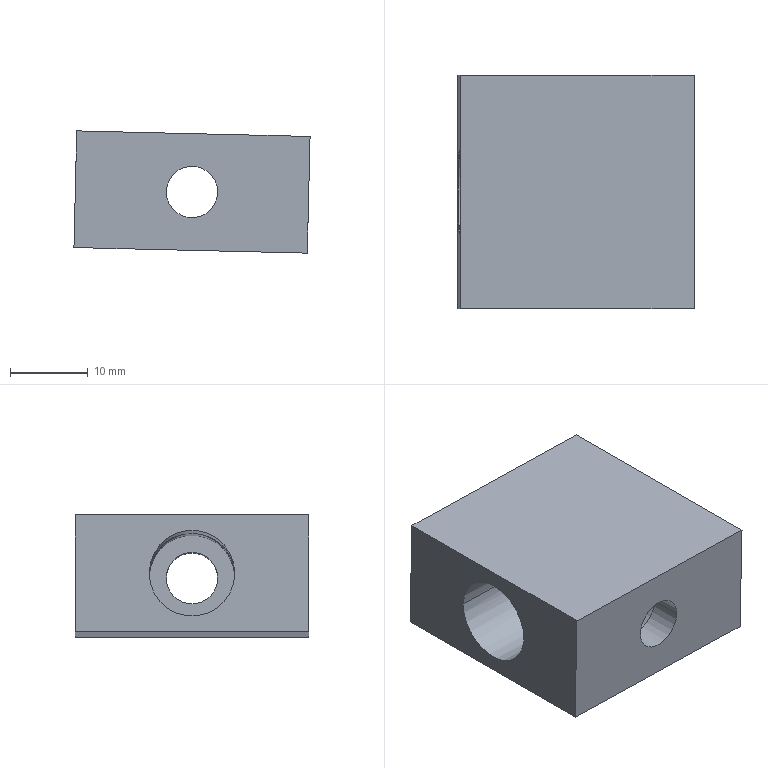Component | SolidWorks | 2012MB0201-1_ASideDoor-1-1_1530ConnectorAMS12-1530-5 | 1 solid | 20 faces | box 30.35 x 30 x 15.71 mm | volume 9172 mm3 | cylinder 12 | plane 8 | commonest cylinder face diameters 11 x8 6.6 x4
build123d program:
from build123d import *

# Parameters (mm, degrees)
SKETCH1_W                                            = 30
SKETCH1_H                                            = 30
BOSS_EXTRUDE1_DEPTH                                  = 15
M6_HEX_SOCKET_HEAD_CAP_SCREW_COUNTERBORE_D           = 6.6
M6_HEX_SOCKET_HEAD_CAP_SCREW_COUNTERBORE_CBORE_D     = 11
M6_HEX_SOCKET_HEAD_CAP_SCREW_COUNTERBORE_CBORE_DEPTH = 26
M6_HEX_SOCKET_HEAD_CAP_SCREW_COUNTER_2_D             = 6.6
M6_HEX_SOCKET_HEAD_CAP_SCREW_COUNTER_2_CBORE_D       = 11
M6_HEX_SOCKET_HEAD_CAP_SCREW_COUNTER_2_CBORE_DEPTH   = 26


with BuildPart() as part:
    # Sketch1 → Boss-Extrude1 (new body)
    with BuildSketch(Plane(origin=(0, 0, 0), x_dir=(1, 0, 0), z_dir=(0, 1, 0))):
        Rectangle(SKETCH1_W, SKETCH1_H)
    extrude(amount=BOSS_EXTRUDE1_DEPTH)

    # M6 Hex Socket Head Cap Screw Counterbore (through all)
    with Locations(Plane(origin=(-15, 7.5, 0), x_dir=(0, 0, -1), z_dir=(-1, 0, 0))):
        with Locations((0, 0)):
            CounterBoreHole(M6_HEX_SOCKET_HEAD_CAP_SCREW_COUNTERBORE_D / 2, M6_HEX_SOCKET_HEAD_CAP_SCREW_COUNTERBORE_CBORE_D / 2, M6_HEX_SOCKET_HEAD_CAP_SCREW_COUNTERBORE_CBORE_DEPTH)

    # M6 Hex Socket Head Cap Screw Counter 2 (through all)
    with Locations(Plane(origin=(0, 7.5, -15), x_dir=(-1, 0, 0), z_dir=(0, 0, -1))):
        with Locations((0, 0)):
            CounterBoreHole(M6_HEX_SOCKET_HEAD_CAP_SCREW_COUNTER_2_D / 2, M6_HEX_SOCKET_HEAD_CAP_SCREW_COUNTER_2_CBORE_D / 2, M6_HEX_SOCKET_HEAD_CAP_SCREW_COUNTER_2_CBORE_DEPTH)


solid = part.part

# Placed as in the assembly
solid = solid.moved(Location((-1264.623, 987.35, -171.755), (-180, 88.629, 90)))
STEP:
#1=COLOUR_RGB('',0.7922,0.8196,0.9333);
#2=FILL_AREA_STYLE_COLOUR('',#1);
#3=FILL_AREA_STYLE('',(#2));
#4=SURFACE_STYLE_FILL_AREA(#3);
#5=SURFACE_SIDE_STYLE('',(#4));
#6=SURFACE_STYLE_USAGE(.BOTH.,#5);
#7=PRESENTATION_STYLE_ASSIGNMENT((#6));
#8=CARTESIAN_POINT('',(-49.205,39.002,-7.071));
#9=VERTEX_POINT('',#8);
#10=CARTESIAN_POINT('',(-49.205,38.742,-7.071));
#11=VERTEX_POINT('',#10);
#12=CARTESIAN_POINT('',(-49.205,38.872,-7.071));
#13=DIRECTION('',(-0.9997,-0.,0.02392));
#14=DIRECTION('',(0.,-1.,0.));
#15=AXIS2_PLACEMENT_3D('',#12,#13,#14);
#16=CIRCLE('',#15,0.1299);
#17=EDGE_CURVE('',#9,#11,#16,.T.);
#18=ORIENTED_EDGE('',*,*,#17,.F.);
#19=CARTESIAN_POINT('',(-49.362,39.002,-7.068));
#20=VERTEX_POINT('',#19);
#21=CARTESIAN_POINT('',(-50.386,39.002,-7.043));
#22=DIRECTION('',(-0.9997,-0.,0.02392));
#23=VECTOR('',#22,39.37);
#24=LINE('',#21,#23);
#25=EDGE_CURVE('',#9,#20,#24,.T.);
#26=ORIENTED_EDGE('',*,*,#25,.T.);
#27=CARTESIAN_POINT('',(-49.362,38.742,-7.068));
#28=VERTEX_POINT('',#27);
#29=CARTESIAN_POINT('',(-49.362,38.872,-7.068));
#30=DIRECTION('',(-0.9997,-0.,0.02392));
#31=DIRECTION('',(0.,-1.,0.));
#32=AXIS2_PLACEMENT_3D('',#29,#30,#31);
#33=CIRCLE('',#32,0.1299);
#34=EDGE_CURVE('',#20,#28,#33,.T.);
#35=ORIENTED_EDGE('',*,*,#34,.T.);
#36=CARTESIAN_POINT('',(-50.386,38.742,-7.043));
#37=DIRECTION('',(-0.9997,-0.,0.02392));
#38=VECTOR('',#37,39.37);
#39=LINE('',#36,#38);
#40=EDGE_CURVE('',#11,#28,#39,.T.);
#41=ORIENTED_EDGE('',*,*,#40,.F.);
#42=EDGE_LOOP('',(#18,#26,#35,#41));
#43=FACE_OUTER_BOUND('',#42,.T.);
#44=CARTESIAN_POINT('',(-50.386,38.872,-7.043));
#45=DIRECTION('',(-0.9997,-0.,0.02392));
#46=DIRECTION('',(0.,-1.,0.));
#47=AXIS2_PLACEMENT_3D('',#44,#45,#46);
#48=CYLINDRICAL_SURFACE('',#47,0.1299);
#49=ADVANCED_FACE('',(#43),#48,.F.);
#50=CARTESIAN_POINT('',(-49.362,39.089,-7.068));
#51=VERTEX_POINT('',#50);
#52=CARTESIAN_POINT('',(-49.362,38.656,-7.068));
#53=VERTEX_POINT('',#52);
#54=CARTESIAN_POINT('',(-49.362,38.872,-7.068));
#55=DIRECTION('',(-0.9997,-0.,0.02392));
#56=DIRECTION('',(0.,-1.,0.));
#57=AXIS2_PLACEMENT_3D('',#54,#55,#56);
#58=CIRCLE('',#57,0.2165);
#59=EDGE_CURVE('',#51,#53,#58,.T.);
#60=ORIENTED_EDGE('',*,*,#59,.F.);
#61=CARTESIAN_POINT('',(-49.579,39.089,-7.062));
#62=VERTEX_POINT('',#61);
#63=CARTESIAN_POINT('',(-50.386,39.089,-7.043));
#64=DIRECTION('',(-0.9997,-0.,0.02392));
#65=VECTOR('',#64,39.37);
#66=LINE('',#63,#65);
#67=EDGE_CURVE('',#51,#62,#66,.T.);
#68=ORIENTED_EDGE('',*,*,#67,.T.);
#69=CARTESIAN_POINT('',(-49.801,38.872,-7.274));
#70=VERTEX_POINT('',#69);
#71=CARTESIAN_POINT('',(-49.801,38.872,-7.274));
#72=CARTESIAN_POINT('',(-49.674,38.999,-7.277));
#73=CARTESIAN_POINT('',(-49.582,39.089,-7.189));
#74=CARTESIAN_POINT('',(-49.579,39.089,-7.062));
#75=(BOUNDED_CURVE()B_SPLINE_CURVE(3,(#71,#72,#73,#74),.UNSPECIFIED.,.F.,.T.)B_SPLINE_CURVE_WITH_KNOTS((4,4),(4.712,6.283),.UNSPECIFIED.)CURVE()GEOMETRIC_REPRESENTATION_ITEM()RATIONAL_B_SPLINE_CURVE((1.,0.8047,0.8047,1.))REPRESENTATION_ITEM(''));
#76=EDGE_CURVE('',#70,#62,#75,.T.);
#77=ORIENTED_EDGE('',*,*,#76,.F.);
#78=CARTESIAN_POINT('',(-49.579,38.656,-7.062));
#79=VERTEX_POINT('',#78);
#80=CARTESIAN_POINT('',(-49.579,38.656,-7.062));
#81=CARTESIAN_POINT('',(-49.582,38.656,-7.189));
#82=CARTESIAN_POINT('',(-49.674,38.745,-7.277));
#83=CARTESIAN_POINT('',(-49.801,38.872,-7.274));
#84=(BOUNDED_CURVE()B_SPLINE_CURVE(3,(#80,#81,#82,#83),.UNSPECIFIED.,.F.,.F.)B_SPLINE_CURVE_WITH_KNOTS((4,4),(3.142,4.712),.UNSPECIFIED.)CURVE()GEOMETRIC_REPRESENTATION_ITEM()RATIONAL_B_SPLINE_CURVE((1.,0.8047,0.8047,1.))REPRESENTATION_ITEM(''));
#85=EDGE_CURVE('',#79,#70,#84,.T.);
#86=ORIENTED_EDGE('',*,*,#85,.F.);
#87=CARTESIAN_POINT('',(-50.386,38.656,-7.043));
#88=DIRECTION('',(-0.9997,-0.,0.02392));
#89=VECTOR('',#88,39.37);
#90=LINE('',#87,#89);
#91=EDGE_CURVE('',#53,#79,#90,.T.);
#92=ORIENTED_EDGE('',*,*,#91,.F.);
#93=EDGE_LOOP('',(#60,#68,#77,#86,#92));
#94=FACE_OUTER_BOUND('',#93,.T.);
#95=CARTESIAN_POINT('',(-50.386,38.872,-7.043));
#96=DIRECTION('',(-0.9997,-0.,0.02392));
#97=DIRECTION('',(0.,-1.,0.));
#98=AXIS2_PLACEMENT_3D('',#95,#96,#97);
#99=CYLINDRICAL_SURFACE('',#98,0.2165);
#100=ADVANCED_FACE('',(#94),#99,.F.);
#101=CARTESIAN_POINT('',(-50.012,39.089,-7.052));
#102=VERTEX_POINT('',#101);
#103=CARTESIAN_POINT('',(-50.012,39.089,-7.052));
#104=CARTESIAN_POINT('',(-50.015,39.089,-7.179));
#105=CARTESIAN_POINT('',(-49.927,38.999,-7.271));
#106=CARTESIAN_POINT('',(-49.801,38.872,-7.274));
#107=(BOUNDED_CURVE()B_SPLINE_CURVE(3,(#103,#104,#105,#106),.UNSPECIFIED.,.F.,.F.)B_SPLINE_CURVE_WITH_KNOTS((4,4),(0.,1.571),.UNSPECIFIED.)CURVE()GEOMETRIC_REPRESENTATION_ITEM()RATIONAL_B_SPLINE_CURVE((1.,0.8047,0.8047,1.))REPRESENTATION_ITEM(''));
#108=EDGE_CURVE('',#102,#70,#107,.T.);
#109=ORIENTED_EDGE('',*,*,#108,.F.);
#110=CARTESIAN_POINT('',(-50.386,39.089,-7.043));
#111=VERTEX_POINT('',#110);
#112=CARTESIAN_POINT('',(-50.386,39.089,-7.043));
#113=DIRECTION('',(-0.9997,-0.,0.02392));
#114=VECTOR('',#113,39.37);
#115=LINE('',#112,#114);
#116=EDGE_CURVE('',#102,#111,#115,.T.);
#117=ORIENTED_EDGE('',*,*,#116,.T.);
#118=CARTESIAN_POINT('',(-50.386,38.656,-7.043));
#119=VERTEX_POINT('',#118);
#120=CARTESIAN_POINT('',(-50.386,38.872,-7.043));
#121=DIRECTION('',(-0.9997,-0.,0.02392));
#122=DIRECTION('',(0.,-1.,0.));
#123=AXIS2_PLACEMENT_3D('',#120,#121,#122);
#124=CIRCLE('',#123,0.2165);
#125=EDGE_CURVE('',#111,#119,#124,.T.);
#126=ORIENTED_EDGE('',*,*,#125,.T.);
#127=CARTESIAN_POINT('',(-50.012,38.656,-7.052));
#128=VERTEX_POINT('',#127);
#129=CARTESIAN_POINT('',(-50.386,38.656,-7.043));
#130=DIRECTION('',(-0.9997,-0.,0.02392));
#131=VECTOR('',#130,39.37);
#132=LINE('',#129,#131);
#133=EDGE_CURVE('',#128,#119,#132,.T.);
#134=ORIENTED_EDGE('',*,*,#133,.F.);
#135=CARTESIAN_POINT('',(-49.801,38.872,-7.274));
#136=CARTESIAN_POINT('',(-49.927,38.745,-7.271));
#137=CARTESIAN_POINT('',(-50.015,38.656,-7.179));
#138=CARTESIAN_POINT('',(-50.012,38.656,-7.052));
#139=(BOUNDED_CURVE()B_SPLINE_CURVE(3,(#135,#136,#137,#138),.UNSPECIFIED.,.F.,.F.)B_SPLINE_CURVE_WITH_KNOTS((4,4),(1.571,3.142),.UNSPECIFIED.)CURVE()GEOMETRIC_REPRESENTATION_ITEM()RATIONAL_B_SPLINE_CURVE((1.,0.8047,0.8047,1.))REPRESENTATION_ITEM(''));
#140=EDGE_CURVE('',#70,#128,#139,.T.);
#141=ORIENTED_EDGE('',*,*,#140,.F.);
#142=EDGE_LOOP('',(#109,#117,#126,#134,#141));
#143=FACE_OUTER_BOUND('',#142,.T.);
#144=CARTESIAN_POINT('',(-50.386,38.872,-7.043));
#145=DIRECTION('',(-0.9997,-0.,0.02392));
#146=DIRECTION('',(0.,-1.,0.));
#147=AXIS2_PLACEMENT_3D('',#144,#145,#146);
#148=CYLINDRICAL_SURFACE('',#147,0.2165);
#149=ADVANCED_FACE('',(#143),#148,.F.);
#150=CARTESIAN_POINT('',(-49.579,38.439,-7.062));
#151=VERTEX_POINT('',#150);
#152=CARTESIAN_POINT('',(-50.012,38.439,-7.052));
#153=VERTEX_POINT('',#152);
#154=CARTESIAN_POINT('',(-49.795,38.439,-7.057));
#155=DIRECTION('',(-0.,1.,0.));
#156=DIRECTION('',(-0.9997,-0.,0.02392));
#157=AXIS2_PLACEMENT_3D('',#154,#155,#156);
#158=CIRCLE('',#157,0.2165);
#159=EDGE_CURVE('',#151,#153,#158,.T.);
#160=ORIENTED_EDGE('',*,*,#159,.F.);
#161=CARTESIAN_POINT('',(-49.579,39.463,-7.062));
#162=DIRECTION('',(-0.,1.,0.));
#163=VECTOR('',#162,39.37);
#164=LINE('',#161,#163);
#165=EDGE_CURVE('',#151,#79,#164,.T.);
#166=ORIENTED_EDGE('',*,*,#165,.T.);
#167=ORIENTED_EDGE('',*,*,#85,.T.);
#168=ORIENTED_EDGE('',*,*,#140,.T.);
#169=CARTESIAN_POINT('',(-50.012,39.463,-7.052));
#170=DIRECTION('',(-0.,1.,0.));
#171=VECTOR('',#170,39.37);
#172=LINE('',#169,#171);
#173=EDGE_CURVE('',#153,#128,#172,.T.);
#174=ORIENTED_EDGE('',*,*,#173,.F.);
#175=EDGE_LOOP('',(#160,#166,#167,#168,#174));
#176=FACE_OUTER_BOUND('',#175,.T.);
#177=CARTESIAN_POINT('',(-49.795,39.463,-7.057));
#178=DIRECTION('',(-0.,1.,0.));
#179=DIRECTION('',(-0.9997,0.,0.02392));
#180=AXIS2_PLACEMENT_3D('',#177,#178,#179);
#181=CYLINDRICAL_SURFACE('',#180,0.2165);
#182=ADVANCED_FACE('',(#176),#181,.F.);
#183=CARTESIAN_POINT('',(-49.666,38.282,-7.06));
#184=VERTEX_POINT('',#183);
#185=CARTESIAN_POINT('',(-49.925,38.282,-7.054));
#186=VERTEX_POINT('',#185);
#187=CARTESIAN_POINT('',(-49.795,38.282,-7.057));
#188=DIRECTION('',(-0.,1.,0.));
#189=DIRECTION('',(-0.9997,0.,0.02392));
#190=AXIS2_PLACEMENT_3D('',#187,#188,#189);
#191=CIRCLE('',#190,0.1299);
#192=EDGE_CURVE('',#184,#186,#191,.T.);
#193=ORIENTED_EDGE('',*,*,#192,.F.);
#194=CARTESIAN_POINT('',(-49.666,38.439,-7.06));
#195=VERTEX_POINT('',#194);
#196=CARTESIAN_POINT('',(-49.666,39.463,-7.06));
#197=DIRECTION('',(-0.,1.,0.));
#198=VECTOR('',#197,39.37);
#199=LINE('',#196,#198);
#200=EDGE_CURVE('',#184,#195,#199,.T.);
#201=ORIENTED_EDGE('',*,*,#200,.T.);
#202=CARTESIAN_POINT('',(-49.925,38.439,-7.054));
#203=VERTEX_POINT('',#202);
#204=CARTESIAN_POINT('',(-49.795,38.439,-7.057));
#205=DIRECTION('',(-0.,1.,0.));
#206=DIRECTION('',(-0.9997,0.,0.02392));
#207=AXIS2_PLACEMENT_3D('',#204,#205,#206);
#208=CIRCLE('',#207,0.1299);
#209=EDGE_CURVE('',#195,#203,#208,.T.);
#210=ORIENTED_EDGE('',*,*,#209,.T.);
#211=CARTESIAN_POINT('',(-49.925,39.463,-7.054));
#212=DIRECTION('',(-0.,1.,0.));
#213=VECTOR('',#212,39.37);
#214=LINE('',#211,#213);
#215=EDGE_CURVE('',#186,#203,#214,.T.);
#216=ORIENTED_EDGE('',*,*,#215,.F.);
#217=EDGE_LOOP('',(#193,#201,#210,#216));
#218=FACE_OUTER_BOUND('',#217,.T.);
#219=CARTESIAN_POINT('',(-49.795,39.463,-7.057));
#220=DIRECTION('',(-0.,1.,0.));
#221=DIRECTION('',(-0.9997,0.,0.02392));
#222=AXIS2_PLACEMENT_3D('',#219,#220,#221);
#223=CYLINDRICAL_SURFACE('',#222,0.1299);
#224=ADVANCED_FACE('',(#218),#223,.F.);
#225=ORIENTED_EDGE('',*,*,#76,.T.);
#226=CARTESIAN_POINT('',(-49.579,39.463,-7.062));
#227=VERTEX_POINT('',#226);
#228=CARTESIAN_POINT('',(-49.579,39.463,-7.062));
#229=DIRECTION('',(-0.,1.,0.));
#230=VECTOR('',#229,39.37);
#231=LINE('',#228,#230);
#232=EDGE_CURVE('',#62,#227,#231,.T.);
#233=ORIENTED_EDGE('',*,*,#232,.T.);
#234=CARTESIAN_POINT('',(-50.012,39.463,-7.052));
#235=VERTEX_POINT('',#234);
#236=CARTESIAN_POINT('',(-49.795,39.463,-7.057));
#237=DIRECTION('',(-0.,1.,0.));
#238=DIRECTION('',(-0.9997,0.,0.02392));
#239=AXIS2_PLACEMENT_3D('',#236,#237,#238);
#240=CIRCLE('',#239,0.2165);
#241=EDGE_CURVE('',#227,#235,#240,.T.);
#242=ORIENTED_EDGE('',*,*,#241,.T.);
#243=CARTESIAN_POINT('',(-50.012,39.463,-7.052));
#244=DIRECTION('',(-0.,1.,0.));
#245=VECTOR('',#244,39.37);
#246=LINE('',#243,#245);
#247=EDGE_CURVE('',#102,#235,#246,.T.);
#248=ORIENTED_EDGE('',*,*,#247,.F.);
#249=ORIENTED_EDGE('',*,*,#108,.T.);
#250=EDGE_LOOP('',(#225,#233,#242,#248,#249));
#251=FACE_OUTER_BOUND('',#250,.T.);
#252=CARTESIAN_POINT('',(-49.795,39.463,-7.057));
#253=DIRECTION('',(-0.,1.,0.));
#254=DIRECTION('',(-0.9997,0.,0.02392));
#255=AXIS2_PLACEMENT_3D('',#252,#253,#254);
#256=CYLINDRICAL_SURFACE('',#255,0.2165);
#257=ADVANCED_FACE('',(#251),#256,.F.);
#258=ORIENTED_EDGE('',*,*,#232,.F.);
#259=CARTESIAN_POINT('',(-49.79,38.872,-6.841));
#260=VERTEX_POINT('',#259);
#261=CARTESIAN_POINT('',(-49.579,39.089,-7.062));
#262=CARTESIAN_POINT('',(-49.576,39.089,-6.936));
#263=CARTESIAN_POINT('',(-49.663,38.999,-6.844));
#264=CARTESIAN_POINT('',(-49.79,38.872,-6.841));
#265=(BOUNDED_CURVE()B_SPLINE_CURVE(3,(#261,#262,#263,#264),.UNSPECIFIED.,.F.,.F.)B_SPLINE_CURVE_WITH_KNOTS((4,4),(0.,1.571),.UNSPECIFIED.)CURVE()GEOMETRIC_REPRESENTATION_ITEM()RATIONAL_B_SPLINE_CURVE((1.,0.8047,0.8047,1.))REPRESENTATION_ITEM(''));
#266=EDGE_CURVE('',#62,#260,#265,.T.);
#267=ORIENTED_EDGE('',*,*,#266,.T.);
#268=CARTESIAN_POINT('',(-49.79,38.872,-6.841));
#269=CARTESIAN_POINT('',(-49.917,38.999,-6.838));
#270=CARTESIAN_POINT('',(-50.009,39.089,-6.925));
#271=CARTESIAN_POINT('',(-50.012,39.089,-7.052));
#272=(BOUNDED_CURVE()B_SPLINE_CURVE(3,(#268,#269,#270,#271),.UNSPECIFIED.,.F.,.F.)B_SPLINE_CURVE_WITH_KNOTS((4,4),(4.712,6.283),.UNSPECIFIED.)CURVE()GEOMETRIC_REPRESENTATION_ITEM()RATIONAL_B_SPLINE_CURVE((1.,0.8047,0.8047,1.))REPRESENTATION_ITEM(''));
#273=EDGE_CURVE('',#260,#102,#272,.T.);
#274=ORIENTED_EDGE('',*,*,#273,.T.);
#275=ORIENTED_EDGE('',*,*,#247,.T.);
#276=CARTESIAN_POINT('',(-49.795,39.463,-7.057));
#277=DIRECTION('',(-0.,1.,0.));
#278=DIRECTION('',(-0.9997,0.,0.02392));
#279=AXIS2_PLACEMENT_3D('',#276,#277,#278);
#280=CIRCLE('',#279,0.2165);
#281=EDGE_CURVE('',#235,#227,#280,.T.);
#282=ORIENTED_EDGE('',*,*,#281,.T.);
#283=EDGE_LOOP('',(#258,#267,#274,#275,#282));
#284=FACE_OUTER_BOUND('',#283,.T.);
#285=CARTESIAN_POINT('',(-49.795,39.463,-7.057));
#286=DIRECTION('',(-0.,1.,0.));
#287=DIRECTION('',(-0.9997,0.,0.02392));
#288=AXIS2_PLACEMENT_3D('',#285,#286,#287);
#289=CYLINDRICAL_SURFACE('',#288,0.2165);
#290=ADVANCED_FACE('',(#284),#289,.F.);
#291=CARTESIAN_POINT('',(-49.205,38.872,-7.071));
#292=DIRECTION('',(-0.9997,-0.,0.02392));
#293=DIRECTION('',(0.,-1.,0.));
#294=AXIS2_PLACEMENT_3D('',#291,#292,#293);
#295=CIRCLE('',#294,0.1299);
#296=EDGE_CURVE('',#11,#9,#295,.T.);
#297=ORIENTED_EDGE('',*,*,#296,.T.);
#298=ORIENTED_EDGE('',*,*,#17,.T.);
#299=EDGE_LOOP('',(#297,#298));
#300=FACE_BOUND('',#299,.T.);
#301=CARTESIAN_POINT('',(-49.212,38.282,-7.367));
#302=VERTEX_POINT('',#301);
#303=CARTESIAN_POINT('',(-49.212,39.463,-7.367));
#304=VERTEX_POINT('',#303);
#305=CARTESIAN_POINT('',(-49.212,39.463,-7.367));
#306=DIRECTION('',(-0.,1.,0.));
#307=VECTOR('',#306,39.37);
#308=LINE('',#305,#307);
#309=EDGE_CURVE('',#302,#304,#308,.T.);
#310=ORIENTED_EDGE('',*,*,#309,.T.);
#311=CARTESIAN_POINT('',(-49.198,39.463,-6.776));
#312=VERTEX_POINT('',#311);
#313=CARTESIAN_POINT('',(-49.198,39.463,-6.776));
#314=DIRECTION('',(-0.02392,0.,-0.9997));
#315=VECTOR('',#314,39.37);
#316=LINE('',#313,#315);
#317=EDGE_CURVE('',#312,#304,#316,.T.);
#318=ORIENTED_EDGE('',*,*,#317,.F.);
#319=CARTESIAN_POINT('',(-49.198,38.282,-6.776));
#320=VERTEX_POINT('',#319);
#321=CARTESIAN_POINT('',(-49.198,39.463,-6.776));
#322=DIRECTION('',(-0.,1.,0.));
#323=VECTOR('',#322,39.37);
#324=LINE('',#321,#323);
#325=EDGE_CURVE('',#320,#312,#324,.T.);
#326=ORIENTED_EDGE('',*,*,#325,.F.);
#327=CARTESIAN_POINT('',(-49.198,38.282,-6.776));
#328=DIRECTION('',(-0.02392,0.,-0.9997));
#329=VECTOR('',#328,39.37);
#330=LINE('',#327,#329);
#331=EDGE_CURVE('',#320,#302,#330,.T.);
#332=ORIENTED_EDGE('',*,*,#331,.T.);
#333=EDGE_LOOP('',(#310,#318,#326,#332));
#334=FACE_OUTER_BOUND('',#333,.T.);
#335=CARTESIAN_POINT('',(-49.198,39.463,-6.776));
#336=DIRECTION('',(-0.9997,-0.,0.02392));
#337=DIRECTION('',(0.,-1.,-0.));
#338=AXIS2_PLACEMENT_3D('',#335,#336,#337);
#339=PLANE('',#338);
#340=ADVANCED_FACE('',(#300,#334),#339,.F.);
#341=ORIENTED_EDGE('',*,*,#281,.F.);
#342=ORIENTED_EDGE('',*,*,#241,.F.);
#343=EDGE_LOOP('',(#341,#342));
#344=FACE_BOUND('',#343,.T.);
#345=CARTESIAN_POINT('',(-50.393,39.463,-7.338));
#346=VERTEX_POINT('',#345);
#347=CARTESIAN_POINT('',(-50.393,39.463,-7.338));
#348=DIRECTION('',(-0.9997,-0.,0.02392));
#349=VECTOR('',#348,39.37);
#350=LINE('',#347,#349);
#351=EDGE_CURVE('',#304,#346,#350,.T.);
#352=ORIENTED_EDGE('',*,*,#351,.T.);
#353=CARTESIAN_POINT('',(-50.379,39.463,-6.748));
#354=VERTEX_POINT('',#353);
#355=CARTESIAN_POINT('',(-50.379,39.463,-6.748));
#356=DIRECTION('',(-0.02392,0.,-0.9997));
#357=VECTOR('',#356,39.37);
#358=LINE('',#355,#357);
#359=EDGE_CURVE('',#354,#346,#358,.T.);
#360=ORIENTED_EDGE('',*,*,#359,.F.);
#361=CARTESIAN_POINT('',(-50.379,39.463,-6.748));
#362=DIRECTION('',(-0.9997,-0.,0.02392));
#363=VECTOR('',#362,39.37);
#364=LINE('',#361,#363);
#365=EDGE_CURVE('',#312,#354,#364,.T.);
#366=ORIENTED_EDGE('',*,*,#365,.F.);
#367=ORIENTED_EDGE('',*,*,#317,.T.);
#368=EDGE_LOOP('',(#352,#360,#366,#367));
#369=FACE_OUTER_BOUND('',#368,.T.);
#370=CARTESIAN_POINT('',(-50.379,39.463,-6.748));
#371=DIRECTION('',(0.,-1.,-0.));
#372=DIRECTION('',(0.9997,0.,-0.02392));
#373=AXIS2_PLACEMENT_3D('',#370,#371,#372);
#374=PLANE('',#373);
#375=ADVANCED_FACE('',(#344,#369),#374,.F.);
#376=CARTESIAN_POINT('',(-50.386,38.872,-7.043));
#377=DIRECTION('',(-0.9997,-0.,0.02392));
#378=DIRECTION('',(0.,-1.,0.));
#379=AXIS2_PLACEMENT_3D('',#376,#377,#378);
#380=CIRCLE('',#379,0.2165);
#381=EDGE_CURVE('',#119,#111,#380,.T.);
#382=ORIENTED_EDGE('',*,*,#381,.F.);
#383=ORIENTED_EDGE('',*,*,#125,.F.);
#384=EDGE_LOOP('',(#382,#383));
#385=FACE_BOUND('',#384,.T.);
#386=CARTESIAN_POINT('',(-50.393,38.282,-7.338));
#387=VERTEX_POINT('',#386);
#388=CARTESIAN_POINT('',(-50.393,39.463,-7.338));
#389=DIRECTION('',(0.,-1.,-0.));
#390=VECTOR('',#389,39.37);
#391=LINE('',#388,#390);
#392=EDGE_CURVE('',#346,#387,#391,.T.);
#393=ORIENTED_EDGE('',*,*,#392,.T.);
#394=CARTESIAN_POINT('',(-50.379,38.282,-6.748));
#395=VERTEX_POINT('',#394);
#396=CARTESIAN_POINT('',(-50.379,38.282,-6.748));
#397=DIRECTION('',(-0.02392,0.,-0.9997));
#398=VECTOR('',#397,39.37);
#399=LINE('',#396,#398);
#400=EDGE_CURVE('',#395,#387,#399,.T.);
#401=ORIENTED_EDGE('',*,*,#400,.F.);
#402=CARTESIAN_POINT('',(-50.379,39.463,-6.748));
#403=DIRECTION('',(0.,-1.,-0.));
#404=VECTOR('',#403,39.37);
#405=LINE('',#402,#404);
#406=EDGE_CURVE('',#354,#395,#405,.T.);
#407=ORIENTED_EDGE('',*,*,#406,.F.);
#408=ORIENTED_EDGE('',*,*,#359,.T.);
#409=EDGE_LOOP('',(#393,#401,#407,#408));
#410=FACE_OUTER_BOUND('',#409,.T.);
#411=CARTESIAN_POINT('',(-50.379,39.463,-6.748));
#412=DIRECTION('',(0.9997,0.,-0.02392));
#413=DIRECTION('',(-0.,1.,0.));
#414=AXIS2_PLACEMENT_3D('',#411,#412,#413);
#415=PLANE('',#414);
#416=ADVANCED_FACE('',(#385,#410),#415,.F.);
#417=CARTESIAN_POINT('',(-49.795,38.282,-7.057));
#418=DIRECTION('',(-0.,1.,0.));
#419=DIRECTION('',(-0.9997,0.,0.02392));
#420=AXIS2_PLACEMENT_3D('',#417,#418,#419);
#421=CIRCLE('',#420,0.1299);
#422=EDGE_CURVE('',#186,#184,#421,.T.);
#423=ORIENTED_EDGE('',*,*,#422,.T.);
#424=ORIENTED_EDGE('',*,*,#192,.T.);
#425=EDGE_LOOP('',(#423,#424));
#426=FACE_BOUND('',#425,.T.);
#427=CARTESIAN_POINT('',(-50.393,38.282,-7.338));
#428=DIRECTION('',(0.9997,0.,-0.02392));
#429=VECTOR('',#428,39.37);
#430=LINE('',#427,#429);
#431=EDGE_CURVE('',#387,#302,#430,.T.);
#432=ORIENTED_EDGE('',*,*,#431,.T.);
#433=ORIENTED_EDGE('',*,*,#331,.F.);
#434=CARTESIAN_POINT('',(-50.379,38.282,-6.748));
#435=DIRECTION('',(0.9997,0.,-0.02392));
#436=VECTOR('',#435,39.37);
#437=LINE('',#434,#436);
#438=EDGE_CURVE('',#395,#320,#437,.T.);
#439=ORIENTED_EDGE('',*,*,#438,.F.);
#440=ORIENTED_EDGE('',*,*,#400,.T.);
#441=EDGE_LOOP('',(#432,#433,#439,#440));
#442=FACE_OUTER_BOUND('',#441,.T.);
#443=CARTESIAN_POINT('',(-50.379,38.282,-6.748));
#444=DIRECTION('',(-0.,1.,0.));
#445=DIRECTION('',(-0.9997,-0.,0.02392));
#446=AXIS2_PLACEMENT_3D('',#443,#444,#445);
#447=PLANE('',#446);
#448=ADVANCED_FACE('',(#426,#442),#447,.F.);
#449=ORIENTED_EDGE('',*,*,#325,.T.);
#450=ORIENTED_EDGE('',*,*,#365,.T.);
#451=ORIENTED_EDGE('',*,*,#406,.T.);
#452=ORIENTED_EDGE('',*,*,#438,.T.);
#453=EDGE_LOOP('',(#449,#450,#451,#452));
#454=FACE_OUTER_BOUND('',#453,.T.);
#455=CARTESIAN_POINT('',(-49.788,38.872,-6.762));
#456=DIRECTION('',(0.02392,-0.,0.9997));
#457=DIRECTION('',(0.,-1.,-0.));
#458=AXIS2_PLACEMENT_3D('',#455,#456,#457);
#459=PLANE('',#458);
#460=ADVANCED_FACE('',(#454),#459,.T.);
#461=ORIENTED_EDGE('',*,*,#309,.F.);
#462=ORIENTED_EDGE('',*,*,#431,.F.);
#463=ORIENTED_EDGE('',*,*,#392,.F.);
#464=ORIENTED_EDGE('',*,*,#351,.F.);
#465=EDGE_LOOP('',(#461,#462,#463,#464));
#466=FACE_OUTER_BOUND('',#465,.T.);
#467=CARTESIAN_POINT('',(-49.802,38.872,-7.352));
#468=DIRECTION('',(0.02392,-0.,0.9997));
#469=DIRECTION('',(0.,-1.,-0.));
#470=AXIS2_PLACEMENT_3D('',#467,#468,#469);
#471=PLANE('',#470);
#472=ADVANCED_FACE('',(#466),#471,.F.);
#473=ORIENTED_EDGE('',*,*,#200,.F.);
#474=ORIENTED_EDGE('',*,*,#422,.F.);
#475=ORIENTED_EDGE('',*,*,#215,.T.);
#476=CARTESIAN_POINT('',(-49.795,38.439,-7.057));
#477=DIRECTION('',(-0.,1.,0.));
#478=DIRECTION('',(-0.9997,0.,0.02392));
#479=AXIS2_PLACEMENT_3D('',#476,#477,#478);
#480=CIRCLE('',#479,0.1299);
#481=EDGE_CURVE('',#203,#195,#480,.T.);
#482=ORIENTED_EDGE('',*,*,#481,.T.);
#483=EDGE_LOOP('',(#473,#474,#475,#482));
#484=FACE_OUTER_BOUND('',#483,.T.);
#485=CARTESIAN_POINT('',(-49.795,39.463,-7.057));
#486=DIRECTION('',(-0.,1.,0.));
#487=DIRECTION('',(-0.9997,0.,0.02392));
#488=AXIS2_PLACEMENT_3D('',#485,#486,#487);
#489=CYLINDRICAL_SURFACE('',#488,0.1299);
#490=ADVANCED_FACE('',(#484),#489,.F.);
#491=ORIENTED_EDGE('',*,*,#481,.F.);
#492=ORIENTED_EDGE('',*,*,#209,.F.);
#493=EDGE_LOOP('',(#491,#492));
#494=FACE_BOUND('',#493,.T.);
#495=CARTESIAN_POINT('',(-49.795,38.439,-7.057));
#496=DIRECTION('',(-0.,1.,0.));
#497=DIRECTION('',(-0.9997,-0.,0.02392));
#498=AXIS2_PLACEMENT_3D('',#495,#496,#497);
#499=CIRCLE('',#498,0.2165);
#500=EDGE_CURVE('',#153,#151,#499,.T.);
#501=ORIENTED_EDGE('',*,*,#500,.T.);
#502=ORIENTED_EDGE('',*,*,#159,.T.);
#503=EDGE_LOOP('',(#501,#502));
#504=FACE_OUTER_BOUND('',#503,.T.);
#505=CARTESIAN_POINT('',(-49.666,38.439,-7.06));
#506=DIRECTION('',(0.,-1.,-0.));
#507=DIRECTION('',(0.9997,0.,-0.02392));
#508=AXIS2_PLACEMENT_3D('',#505,#506,#507);
#509=PLANE('',#508);
#510=ADVANCED_FACE('',(#494,#504),#509,.F.);
#511=ORIENTED_EDGE('',*,*,#165,.F.);
#512=ORIENTED_EDGE('',*,*,#500,.F.);
#513=ORIENTED_EDGE('',*,*,#173,.T.);
#514=CARTESIAN_POINT('',(-50.012,38.656,-7.052));
#515=CARTESIAN_POINT('',(-50.009,38.656,-6.925));
#516=CARTESIAN_POINT('',(-49.917,38.745,-6.838));
#517=CARTESIAN_POINT('',(-49.79,38.872,-6.841));
#518=(BOUNDED_CURVE()B_SPLINE_CURVE(3,(#514,#515,#516,#517),.UNSPECIFIED.,.F.,.F.)B_SPLINE_CURVE_WITH_KNOTS((4,4),(3.142,4.712),.UNSPECIFIED.)CURVE()GEOMETRIC_REPRESENTATION_ITEM()RATIONAL_B_SPLINE_CURVE((1.,0.8047,0.8047,1.))REPRESENTATION_ITEM(''));
#519=EDGE_CURVE('',#128,#260,#518,.T.);
#520=ORIENTED_EDGE('',*,*,#519,.T.);
#521=CARTESIAN_POINT('',(-49.79,38.872,-6.841));
#522=CARTESIAN_POINT('',(-49.663,38.745,-6.844));
#523=CARTESIAN_POINT('',(-49.576,38.656,-6.936));
#524=CARTESIAN_POINT('',(-49.579,38.656,-7.062));
#525=(BOUNDED_CURVE()B_SPLINE_CURVE(3,(#521,#522,#523,#524),.UNSPECIFIED.,.F.,.F.)B_SPLINE_CURVE_WITH_KNOTS((4,4),(1.571,3.142),.UNSPECIFIED.)CURVE()GEOMETRIC_REPRESENTATION_ITEM()RATIONAL_B_SPLINE_CURVE((1.,0.8047,0.8047,1.))REPRESENTATION_ITEM(''));
#526=EDGE_CURVE('',#260,#79,#525,.T.);
#527=ORIENTED_EDGE('',*,*,#526,.T.);
#528=EDGE_LOOP('',(#511,#512,#513,#520,#527));
#529=FACE_OUTER_BOUND('',#528,.T.);
#530=CARTESIAN_POINT('',(-49.795,39.463,-7.057));
#531=DIRECTION('',(-0.,1.,0.));
#532=DIRECTION('',(-0.9997,0.,0.02392));
#533=AXIS2_PLACEMENT_3D('',#530,#531,#532);
#534=CYLINDRICAL_SURFACE('',#533,0.2165);
#535=ADVANCED_FACE('',(#529),#534,.F.);
#536=ORIENTED_EDGE('',*,*,#116,.F.);
#537=ORIENTED_EDGE('',*,*,#273,.F.);
#538=ORIENTED_EDGE('',*,*,#519,.F.);
#539=ORIENTED_EDGE('',*,*,#133,.T.);
#540=ORIENTED_EDGE('',*,*,#381,.T.);
#541=EDGE_LOOP('',(#536,#537,#538,#539,#540));
#542=FACE_OUTER_BOUND('',#541,.T.);
#543=CARTESIAN_POINT('',(-50.386,38.872,-7.043));
#544=DIRECTION('',(-0.9997,-0.,0.02392));
#545=DIRECTION('',(0.,-1.,0.));
#546=AXIS2_PLACEMENT_3D('',#543,#544,#545);
#547=CYLINDRICAL_SURFACE('',#546,0.2165);
#548=ADVANCED_FACE('',(#542),#547,.F.);
#549=ORIENTED_EDGE('',*,*,#67,.F.);
#550=CARTESIAN_POINT('',(-49.362,38.872,-7.068));
#551=DIRECTION('',(-0.9997,-0.,0.02392));
#552=DIRECTION('',(0.,-1.,0.));
#553=AXIS2_PLACEMENT_3D('',#550,#551,#552);
#554=CIRCLE('',#553,0.2165);
#555=EDGE_CURVE('',#53,#51,#554,.T.);
#556=ORIENTED_EDGE('',*,*,#555,.F.);
#557=ORIENTED_EDGE('',*,*,#91,.T.);
#558=ORIENTED_EDGE('',*,*,#526,.F.);
#559=ORIENTED_EDGE('',*,*,#266,.F.);
#560=EDGE_LOOP('',(#549,#556,#557,#558,#559));
#561=FACE_OUTER_BOUND('',#560,.T.);
#562=CARTESIAN_POINT('',(-50.386,38.872,-7.043));
#563=DIRECTION('',(-0.9997,-0.,0.02392));
#564=DIRECTION('',(0.,-1.,0.));
#565=AXIS2_PLACEMENT_3D('',#562,#563,#564);
#566=CYLINDRICAL_SURFACE('',#565,0.2165);
#567=ADVANCED_FACE('',(#561),#566,.F.);
#568=ORIENTED_EDGE('',*,*,#25,.F.);
#569=ORIENTED_EDGE('',*,*,#296,.F.);
#570=ORIENTED_EDGE('',*,*,#40,.T.);
#571=CARTESIAN_POINT('',(-49.362,38.872,-7.068));
#572=DIRECTION('',(-0.9997,-0.,0.02392));
#573=DIRECTION('',(0.,-1.,0.));
#574=AXIS2_PLACEMENT_3D('',#571,#572,#573);
#575=CIRCLE('',#574,0.1299);
#576=EDGE_CURVE('',#28,#20,#575,.T.);
#577=ORIENTED_EDGE('',*,*,#576,.T.);
#578=EDGE_LOOP('',(#568,#569,#570,#577));
#579=FACE_OUTER_BOUND('',#578,.T.);
#580=CARTESIAN_POINT('',(-50.386,38.872,-7.043));
#581=DIRECTION('',(-0.9997,-0.,0.02392));
#582=DIRECTION('',(0.,-1.,0.));
#583=AXIS2_PLACEMENT_3D('',#580,#581,#582);
#584=CYLINDRICAL_SURFACE('',#583,0.1299);
#585=ADVANCED_FACE('',(#579),#584,.F.);
#586=ORIENTED_EDGE('',*,*,#576,.F.);
#587=ORIENTED_EDGE('',*,*,#34,.F.);
#588=EDGE_LOOP('',(#586,#587));
#589=FACE_BOUND('',#588,.T.);
#590=ORIENTED_EDGE('',*,*,#555,.T.);
#591=ORIENTED_EDGE('',*,*,#59,.T.);
#592=EDGE_LOOP('',(#590,#591));
#593=FACE_OUTER_BOUND('',#592,.T.);
#594=CARTESIAN_POINT('',(-49.359,38.872,-6.938));
#595=DIRECTION('',(0.9997,0.,-0.02392));
#596=DIRECTION('',(-0.,1.,0.));
#597=AXIS2_PLACEMENT_3D('',#594,#595,#596);
#598=PLANE('',#597);
#599=ADVANCED_FACE('',(#589,#593),#598,.F.);
#600=CLOSED_SHELL('',(#49,#100,#149,#182,#224,#257,#290,#340,#375,#416,#448,#460,#472,#490,#510,#535,#548,#567,#585,#599));
#601=MANIFOLD_SOLID_BREP('',#600);
#602=STYLED_ITEM('',(#7),#601);
#603=PRESENTATION_LAYER_ASSIGNMENT('','',(#602));
#604=CARTESIAN_POINT('',(0.,0.,0.));
#605=DIRECTION('',(0.,0.,1.));
#606=DIRECTION('',(1.,0.,0.));
#607=AXIS2_PLACEMENT_3D('',#604,#605,#606);
#608=(LENGTH_UNIT()NAMED_UNIT(*)SI_UNIT($,.METRE.));
#609=LENGTH_MEASURE_WITH_UNIT(LENGTH_MEASURE(0.0254),#608);
#610=DIMENSIONAL_EXPONENTS(1.,0.,0.,0.,0.,0.,0.);
#611=(CONVERSION_BASED_UNIT('',#609)LENGTH_UNIT()NAMED_UNIT(#610));
#612=UNCERTAINTY_MEASURE_WITH_UNIT(LENGTH_MEASURE(0.00001),#611,'','');
#613=(NAMED_UNIT(*)PLANE_ANGLE_UNIT()SI_UNIT($,.RADIAN.));
#614=(NAMED_UNIT(*)SI_UNIT($,.STERADIAN.)SOLID_ANGLE_UNIT());
#615=(GEOMETRIC_REPRESENTATION_CONTEXT(3)GLOBAL_UNCERTAINTY_ASSIGNED_CONTEXT((#612))GLOBAL_UNIT_ASSIGNED_CONTEXT((#611,#613,#614))REPRESENTATION_CONTEXT('',''));
#616=ADVANCED_BREP_SHAPE_REPRESENTATION('',(#601,#607),#615);
#617=(LENGTH_UNIT()NAMED_UNIT(*)SI_UNIT($,.METRE.));
#618=LENGTH_MEASURE_WITH_UNIT(LENGTH_MEASURE(0.0254),#617);
#619=DIMENSIONAL_EXPONENTS(1.,0.,0.,0.,0.,0.,0.);
#620=(CONVERSION_BASED_UNIT('',#618)LENGTH_UNIT()NAMED_UNIT(#619));
#621=UNCERTAINTY_MEASURE_WITH_UNIT(LENGTH_MEASURE(0.00001),#620,'','');
#622=(NAMED_UNIT(*)PLANE_ANGLE_UNIT()SI_UNIT($,.RADIAN.));
#623=(NAMED_UNIT(*)SI_UNIT($,.STERADIAN.)SOLID_ANGLE_UNIT());
#624=(GEOMETRIC_REPRESENTATION_CONTEXT(3)GLOBAL_UNCERTAINTY_ASSIGNED_CONTEXT((#621))GLOBAL_UNIT_ASSIGNED_CONTEXT((#620,#622,#623))REPRESENTATION_CONTEXT('',''));
#625=MECHANICAL_DESIGN_GEOMETRIC_PRESENTATION_REPRESENTATION('',(#602),#624);